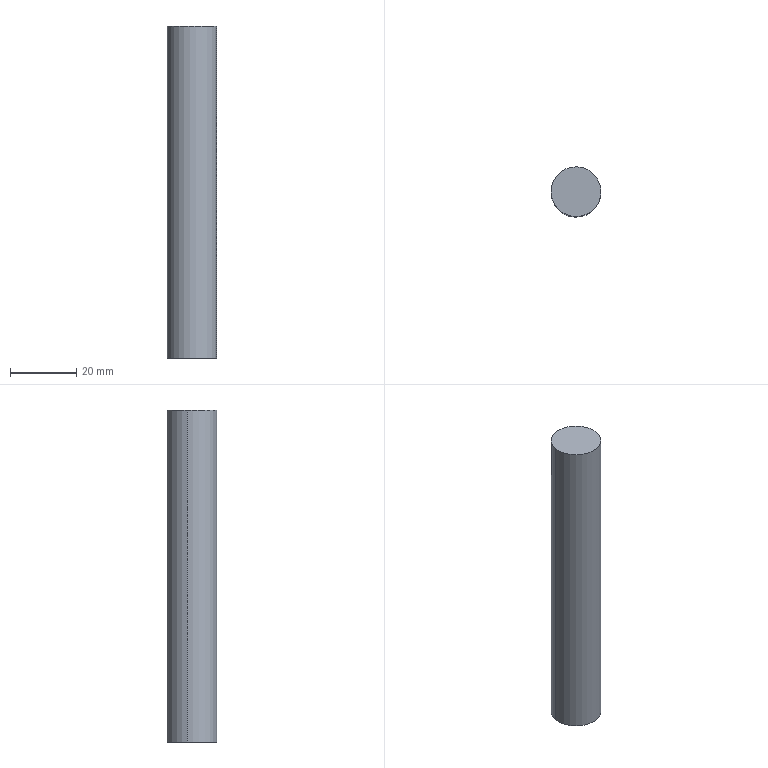Component | SolidWorks | 2023-12-12-31-1 | 1 solid | 4 faces | box 15 x 15 x 100 mm | volume 17671 mm3 | cylinder 2 | plane 2 | commonest cylinder face diameters 15 x2
build123d program:
from build123d import *

# Parameters (mm, degrees)
SKETCH1_R           = 7.5
BOSS_EXTRUDE1_DEPTH = 100


with BuildPart() as part:
    # Sketch1 → Boss-Extrude1 (new body)
    with BuildSketch(Plane.XY):
        Circle(SKETCH1_R)
    extrude(amount=BOSS_EXTRUDE1_DEPTH)


solid = part.part

# Placed as in the assembly
solid = solid.moved(Location((91.222, 67.133, -19), (0, 0, 0)))
STEP:
#1=COLOUR_RGB('',0.7922,0.8196,0.9333);
#2=FILL_AREA_STYLE_COLOUR('',#1);
#3=FILL_AREA_STYLE('',(#2));
#4=SURFACE_STYLE_FILL_AREA(#3);
#5=SURFACE_SIDE_STYLE('',(#4));
#6=SURFACE_STYLE_USAGE(.BOTH.,#5);
#7=PRESENTATION_STYLE_ASSIGNMENT((#6));
#8=CARTESIAN_POINT('',(3.882,2.588,3.189));
#9=VERTEX_POINT('',#8);
#10=CARTESIAN_POINT('',(3.301,2.698,3.189));
#11=VERTEX_POINT('',#10);
#12=CARTESIAN_POINT('',(3.591,2.643,3.189));
#13=DIRECTION('',(0.,0.,1.));
#14=DIRECTION('',(0.9826,-0.1858,0.));
#15=AXIS2_PLACEMENT_3D('',#12,#13,#14);
#16=CIRCLE('',#15,0.2953);
#17=EDGE_CURVE('',#9,#11,#16,.T.);
#18=ORIENTED_EDGE('',*,*,#17,.F.);
#19=CARTESIAN_POINT('',(3.882,2.588,-0.748));
#20=VERTEX_POINT('',#19);
#21=CARTESIAN_POINT('',(3.882,2.588,3.189));
#22=DIRECTION('',(0.,0.,-1.));
#23=VECTOR('',#22,39.37);
#24=LINE('',#21,#23);
#25=EDGE_CURVE('',#9,#20,#24,.T.);
#26=ORIENTED_EDGE('',*,*,#25,.T.);
#27=CARTESIAN_POINT('',(3.301,2.698,-0.748));
#28=VERTEX_POINT('',#27);
#29=CARTESIAN_POINT('',(3.591,2.643,-0.748));
#30=DIRECTION('',(0.,0.,1.));
#31=DIRECTION('',(0.9826,-0.1858,0.));
#32=AXIS2_PLACEMENT_3D('',#29,#30,#31);
#33=CIRCLE('',#32,0.2953);
#34=EDGE_CURVE('',#20,#28,#33,.T.);
#35=ORIENTED_EDGE('',*,*,#34,.T.);
#36=CARTESIAN_POINT('',(3.301,2.698,3.189));
#37=DIRECTION('',(0.,0.,-1.));
#38=VECTOR('',#37,39.37);
#39=LINE('',#36,#38);
#40=EDGE_CURVE('',#11,#28,#39,.T.);
#41=ORIENTED_EDGE('',*,*,#40,.F.);
#42=EDGE_LOOP('',(#18,#26,#35,#41));
#43=FACE_OUTER_BOUND('',#42,.T.);
#44=CARTESIAN_POINT('',(3.591,2.643,3.189));
#45=DIRECTION('',(0.,0.,-1.));
#46=DIRECTION('',(-0.9826,0.1858,0.));
#47=AXIS2_PLACEMENT_3D('',#44,#45,#46);
#48=CYLINDRICAL_SURFACE('',#47,0.2953);
#49=ADVANCED_FACE('',(#43),#48,.T.);
#50=ORIENTED_EDGE('',*,*,#25,.F.);
#51=CARTESIAN_POINT('',(3.591,2.643,3.189));
#52=DIRECTION('',(0.,0.,1.));
#53=DIRECTION('',(0.9826,-0.1858,0.));
#54=AXIS2_PLACEMENT_3D('',#51,#52,#53);
#55=CIRCLE('',#54,0.2953);
#56=EDGE_CURVE('',#11,#9,#55,.T.);
#57=ORIENTED_EDGE('',*,*,#56,.F.);
#58=ORIENTED_EDGE('',*,*,#40,.T.);
#59=CARTESIAN_POINT('',(3.591,2.643,-0.748));
#60=DIRECTION('',(0.,0.,1.));
#61=DIRECTION('',(0.9826,-0.1858,0.));
#62=AXIS2_PLACEMENT_3D('',#59,#60,#61);
#63=CIRCLE('',#62,0.2953);
#64=EDGE_CURVE('',#28,#20,#63,.T.);
#65=ORIENTED_EDGE('',*,*,#64,.T.);
#66=EDGE_LOOP('',(#50,#57,#58,#65));
#67=FACE_OUTER_BOUND('',#66,.T.);
#68=CARTESIAN_POINT('',(3.591,2.643,3.189));
#69=DIRECTION('',(0.,0.,-1.));
#70=DIRECTION('',(-0.9826,0.1858,0.));
#71=AXIS2_PLACEMENT_3D('',#68,#69,#70);
#72=CYLINDRICAL_SURFACE('',#71,0.2953);
#73=ADVANCED_FACE('',(#67),#72,.T.);
#74=ORIENTED_EDGE('',*,*,#56,.T.);
#75=ORIENTED_EDGE('',*,*,#17,.T.);
#76=EDGE_LOOP('',(#74,#75));
#77=FACE_OUTER_BOUND('',#76,.T.);
#78=CARTESIAN_POINT('',(3.591,2.643,3.189));
#79=DIRECTION('',(0.,0.,1.));
#80=DIRECTION('',(0.9826,-0.1858,0.));
#81=AXIS2_PLACEMENT_3D('',#78,#79,#80);
#82=PLANE('',#81);
#83=ADVANCED_FACE('',(#77),#82,.T.);
#84=ORIENTED_EDGE('',*,*,#64,.F.);
#85=ORIENTED_EDGE('',*,*,#34,.F.);
#86=EDGE_LOOP('',(#84,#85));
#87=FACE_OUTER_BOUND('',#86,.T.);
#88=CARTESIAN_POINT('',(3.591,2.643,-0.748));
#89=DIRECTION('',(0.,0.,1.));
#90=DIRECTION('',(0.9826,-0.1858,0.));
#91=AXIS2_PLACEMENT_3D('',#88,#89,#90);
#92=PLANE('',#91);
#93=ADVANCED_FACE('',(#87),#92,.F.);
#94=CLOSED_SHELL('',(#49,#73,#83,#93));
#95=MANIFOLD_SOLID_BREP('',#94);
#96=STYLED_ITEM('',(#7),#95);
#97=(LENGTH_UNIT()NAMED_UNIT(*)SI_UNIT($,.METRE.));
#98=LENGTH_MEASURE_WITH_UNIT(LENGTH_MEASURE(0.0254),#97);
#99=DIMENSIONAL_EXPONENTS(1.,0.,0.,0.,0.,0.,0.);
#100=(CONVERSION_BASED_UNIT('',#98)LENGTH_UNIT()NAMED_UNIT(#99));
#101=UNCERTAINTY_MEASURE_WITH_UNIT(LENGTH_MEASURE(0.00001),#100,'','');
#102=(NAMED_UNIT(*)PLANE_ANGLE_UNIT()SI_UNIT($,.RADIAN.));
#103=(NAMED_UNIT(*)SI_UNIT($,.STERADIAN.)SOLID_ANGLE_UNIT());
#104=(GEOMETRIC_REPRESENTATION_CONTEXT(3)GLOBAL_UNCERTAINTY_ASSIGNED_CONTEXT((#101))GLOBAL_UNIT_ASSIGNED_CONTEXT((#100,#102,#103))REPRESENTATION_CONTEXT('',''));
#105=MECHANICAL_DESIGN_GEOMETRIC_PRESENTATION_REPRESENTATION('',(#96),#104);
#106=PRESENTATION_LAYER_ASSIGNMENT('','',(#96));
#107=CARTESIAN_POINT('',(0.,0.,0.));
#108=DIRECTION('',(0.,0.,1.));
#109=DIRECTION('',(1.,0.,0.));
#110=AXIS2_PLACEMENT_3D('',#107,#108,#109);
#111=(LENGTH_UNIT()NAMED_UNIT(*)SI_UNIT($,.METRE.));
#112=LENGTH_MEASURE_WITH_UNIT(LENGTH_MEASURE(0.0254),#111);
#113=DIMENSIONAL_EXPONENTS(1.,0.,0.,0.,0.,0.,0.);
#114=(CONVERSION_BASED_UNIT('',#112)LENGTH_UNIT()NAMED_UNIT(#113));
#115=UNCERTAINTY_MEASURE_WITH_UNIT(LENGTH_MEASURE(0.00001),#114,'','');
#116=(NAMED_UNIT(*)PLANE_ANGLE_UNIT()SI_UNIT($,.RADIAN.));
#117=(NAMED_UNIT(*)SI_UNIT($,.STERADIAN.)SOLID_ANGLE_UNIT());
#118=(GEOMETRIC_REPRESENTATION_CONTEXT(3)GLOBAL_UNCERTAINTY_ASSIGNED_CONTEXT((#115))GLOBAL_UNIT_ASSIGNED_CONTEXT((#114,#116,#117))REPRESENTATION_CONTEXT('',''));
#119=ADVANCED_BREP_SHAPE_REPRESENTATION('',(#95,#110),#118);